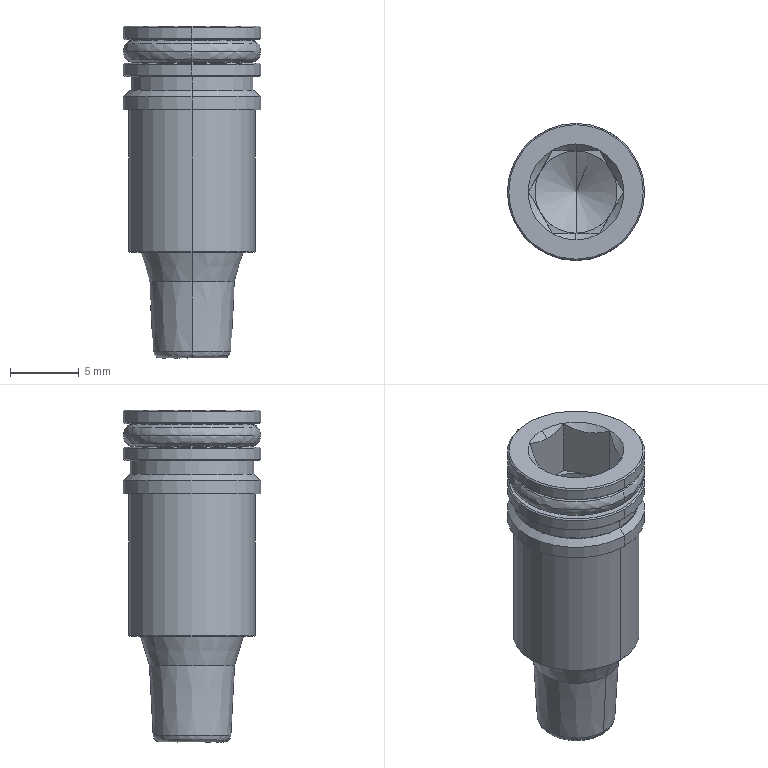Component | SolidWorks | SC-80x75(000)-1_12-1 | 1 solid | 70 faces | volume 1196 mm3 | cone 20 | plane 20 | cylinder 16 | spline 14 | commonest cylinder face diameters 10 x6 7.7 x4 9.188 x2 9 x2 6 x2